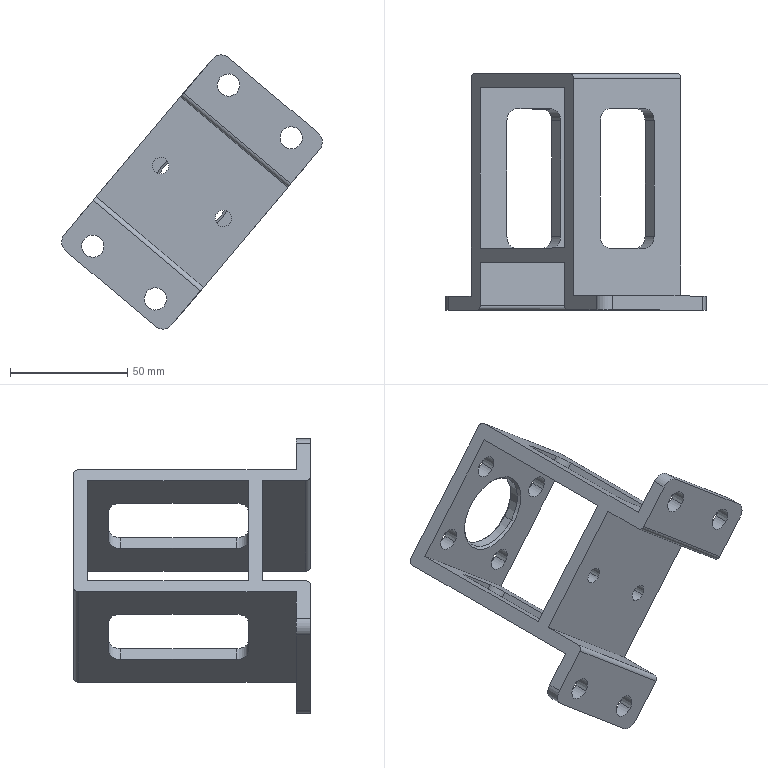Component | SolidWorks | 07FixtureBase-1 | 1 solid | 66 faces | box 111.37 x 101 x 117.17 mm | volume 97150 mm3 | cylinder 38 | plane 24 | cone 4 | commonest cylinder face diameters 9.5 x16 10 x12 7 x4 4 x4 32 x2 | material Aviation Aluminum-7075
build123d program:
from build123d import *

# Parameters (mm, degrees)
BOSS_EXTRUDE1_DEPTH       = 60
CUT_EXTRUDE1_REACH        = 161.578
SKETCH2_R                 = 4.75
CUT_EXTRUDE2_REACH        = 157.849
SKETCH3_R                 = 4.75
FILLET1_R                 = 5
CUT_EXTRUDE3_REACH        = 157.849
SKETCH4_R                 = 16
CUT_EXTRUDE4_DEPTH        = 147.782
BOSS_EXTRUDE2_REACH       = 145.265
SKETCH6_W                 = 60
SKETCH6_H                 = 6
M8X1_0_TAPPED_HOLE1_D     = 7
M8X1_0_TAPPED_HOLE1_DEPTH = 19
M8X1_0_TAPPED_HOLE1_TIP   = 2.103
FILLET2_R                 = 2
CHAMFER1_SIZE             = 1
FILLET3_R                 = 2


with BuildPart() as part:
    # Sketch1 → Boss-Extrude1 (new body)
    with BuildSketch(Plane.XY):
        Polygon((0, 0), (26, 0), (26, -95), (82, -95), (82, 0), (108, 0), (108, -6), (88, -6), (88, -101), (20, -101), (20, -6), (0, -6), align=None)
    extrude(amount=BOSS_EXTRUDE1_DEPTH)

    # Sketch2 → Cut-Extrude1 (cut, up to next)
    with BuildSketch(Plane(origin=(0, 0, 0), x_dir=(1, 0, 0), z_dir=(0, 1, 0)), mode=Mode.PRIVATE) as cut_extrude1_sk1:
        with Locations(Location((9, -12.5, 0), (0, 0, 270))):
            Circle(SKETCH2_R)
    cut_extrude1_tool1 = extrude(cut_extrude1_sk1.sketch, amount=-CUT_EXTRUDE1_REACH, mode=Mode.PRIVATE) & part.part
    # Sketch2 → Cut-Extrude1 (cut, up to next)
    with BuildSketch(Plane(origin=(0, 0, 0), x_dir=(1, 0, 0), z_dir=(0, 1, 0)), mode=Mode.PRIVATE) as cut_extrude1_sk2:
        with Locations(Location((9, -47.5, 0), (0, 0, 270))):
            Circle(SKETCH2_R)
    cut_extrude1_tool2 = extrude(cut_extrude1_sk2.sketch, amount=-CUT_EXTRUDE1_REACH, mode=Mode.PRIVATE) & part.part
    # Sketch2 → Cut-Extrude1 (cut, up to next)
    with BuildSketch(Plane(origin=(0, 0, 0), x_dir=(1, 0, 0), z_dir=(0, 1, 0)), mode=Mode.PRIVATE) as cut_extrude1_sk3:
        with Locations(Location((99, -12.5, 0), (0, 0, 270))):
            Circle(SKETCH2_R)
    cut_extrude1_tool3 = extrude(cut_extrude1_sk3.sketch, amount=-CUT_EXTRUDE1_REACH, mode=Mode.PRIVATE) & part.part
    # Sketch2 → Cut-Extrude1 (cut, up to next)
    with BuildSketch(Plane(origin=(0, 0, 0), x_dir=(1, 0, 0), z_dir=(0, 1, 0)), mode=Mode.PRIVATE) as cut_extrude1_sk4:
        with Locations(Location((99, -47.5, 0), (0, 0, 270))):
            Circle(SKETCH2_R)
    cut_extrude1_tool4 = extrude(cut_extrude1_sk4.sketch, amount=-CUT_EXTRUDE1_REACH, mode=Mode.PRIVATE) & part.part
    add(cut_extrude1_tool1.solids().sort_by_distance((9, 0, 12.5))[0], mode=Mode.SUBTRACT)
    add(cut_extrude1_tool2.solids().sort_by_distance((9, 0, 47.5))[0], mode=Mode.SUBTRACT)
    add(cut_extrude1_tool3.solids().sort_by_distance((99, 0, 12.5))[0], mode=Mode.SUBTRACT)
    add(cut_extrude1_tool4.solids().sort_by_distance((99, 0, 47.5))[0], mode=Mode.SUBTRACT)

    # Sketch3 → Cut-Extrude2 (cut, up to next)
    with BuildSketch(Plane(origin=(0, -95, 0), x_dir=(1, 0, 0), z_dir=(0, 1, 0)), mode=Mode.PRIVATE) as cut_extrude2_sk1:
        with Locations(Location((36.5, -10, 0), (0, 0, 270))):
            Circle(SKETCH3_R)
    cut_extrude2_tool1 = extrude(cut_extrude2_sk1.sketch, amount=-CUT_EXTRUDE2_REACH, mode=Mode.PRIVATE) & part.part
    # Sketch3 → Cut-Extrude2 (cut, up to next)
    with BuildSketch(Plane(origin=(0, -95, 0), x_dir=(1, 0, 0), z_dir=(0, 1, 0)), mode=Mode.PRIVATE) as cut_extrude2_sk2:
        with Locations(Location((71.5, -10, 0), (0, 0, 270))):
            Circle(SKETCH3_R)
    cut_extrude2_tool2 = extrude(cut_extrude2_sk2.sketch, amount=-CUT_EXTRUDE2_REACH, mode=Mode.PRIVATE) & part.part
    # Sketch3 → Cut-Extrude2 (cut, up to next)
    with BuildSketch(Plane(origin=(0, -95, 0), x_dir=(1, 0, 0), z_dir=(0, 1, 0)), mode=Mode.PRIVATE) as cut_extrude2_sk3:
        with Locations(Location((36.5, -50, 0), (0, 0, 270))):
            Circle(SKETCH3_R)
    cut_extrude2_tool3 = extrude(cut_extrude2_sk3.sketch, amount=-CUT_EXTRUDE2_REACH, mode=Mode.PRIVATE) & part.part
    # Sketch3 → Cut-Extrude2 (cut, up to next)
    with BuildSketch(Plane(origin=(0, -95, 0), x_dir=(1, 0, 0), z_dir=(0, 1, 0)), mode=Mode.PRIVATE) as cut_extrude2_sk4:
        with Locations(Location((71.5, -50, 0), (0, 0, 270))):
            Circle(SKETCH3_R)
    cut_extrude2_tool4 = extrude(cut_extrude2_sk4.sketch, amount=-CUT_EXTRUDE2_REACH, mode=Mode.PRIVATE) & part.part
    add(cut_extrude2_tool1.solids().sort_by_distance((36.5, -95, 10))[0], mode=Mode.SUBTRACT)
    add(cut_extrude2_tool2.solids().sort_by_distance((71.5, -95, 10))[0], mode=Mode.SUBTRACT)
    add(cut_extrude2_tool3.solids().sort_by_distance((36.5, -95, 50))[0], mode=Mode.SUBTRACT)
    add(cut_extrude2_tool4.solids().sort_by_distance((71.5, -95, 50))[0], mode=Mode.SUBTRACT)

    # Fillet1
    fillet1_edges = [part.edges().sort_by_distance(p)[0] for p in [
        (108, -3, 0),
        (0, -3, 0),
        (108, -3, 60),
        (0, -3, 60),
    ]]
    fillet(fillet1_edges, radius=FILLET1_R)

    # Sketch4 → Cut-Extrude3 (cut, up to next)
    with BuildSketch(Plane(origin=(0, -95, 0), x_dir=(1, 0, 0), z_dir=(0, 1, 0)), mode=Mode.PRIVATE) as cut_extrude3_sk1:
        with Locations(Location((54, -30, 0), (0, 0, 270))):
            Circle(SKETCH4_R)
    cut_extrude3_tool1 = extrude(cut_extrude3_sk1.sketch, amount=-CUT_EXTRUDE3_REACH, mode=Mode.PRIVATE) & part.part
    add(cut_extrude3_tool1.solids().sort_by_distance((54, -95, 30))[0], mode=Mode.SUBTRACT)

    # Sketch5 → Cut-Extrude4 (cut, through all)
    with BuildSketch(Plane(origin=(88, 0, 0), x_dir=(0, 0, -1), z_dir=(1, 0, 0))):
        with BuildLine():
            Line((-20, -26.5), (-40, -26.5))
            ThreePointArc((-40, -26.5), (-43.536, -27.964), (-45, -31.5))
            Line((-45, -31.5), (-45, -81))
            ThreePointArc((-45, -81), (-43.536, -84.536), (-40, -86))
            Line((-40, -86), (-20, -86))
            ThreePointArc((-20, -86), (-16.464, -84.536), (-15, -81))
            Line((-15, -81), (-15, -31.5))
            ThreePointArc((-15, -31.5), (-16.464, -27.964), (-20, -26.5))
        make_face()
    extrude(amount=-CUT_EXTRUDE4_DEPTH, mode=Mode.SUBTRACT)

    # Sketch6 → Boss-Extrude2 (add, up to next)
    with BuildSketch(Plane(origin=(26, 0, 0), x_dir=(0, 0, -1), z_dir=(1, 0, 0)), mode=Mode.PRIVATE) as boss_extrude2_sk1:
        with Locations((-30, -23.5)):
            Rectangle(SKETCH6_W, SKETCH6_H)
    boss_extrude2_tool1 = extrude(boss_extrude2_sk1.sketch, amount=BOSS_EXTRUDE2_REACH, mode=Mode.PRIVATE) - part.part
    add(boss_extrude2_tool1.solids().sort_by_distance((26, -23.5, 30))[0])

    # M8x1.0 Tapped Hole1
    with Locations(Plane(origin=(54, -20.5, 12.5), x_dir=(1, 0, 0), z_dir=(0, 1, 0))):
        with Locations((0, 0), (0, -35)):
            Hole(M8X1_0_TAPPED_HOLE1_D / 2, depth=M8X1_0_TAPPED_HOLE1_DEPTH)
            with Locations((0, 0, -(M8X1_0_TAPPED_HOLE1_DEPTH + M8X1_0_TAPPED_HOLE1_TIP / 2))):  # 118° drill point
                Cone(0, M8X1_0_TAPPED_HOLE1_D / 2, M8X1_0_TAPPED_HOLE1_TIP, mode=Mode.SUBTRACT)

    # Fillet2
    fillet2_edges = [part.edges().sort_by_distance(p)[0] for p in [
        (88, -101, 30),
        (20, -101, 30),
    ]]
    fillet(fillet2_edges, radius=FILLET2_R)

    # Chamfer1
    chamfer1_edges = [part.edges().sort_by_distance(p)[0] for p in [
        (54, -95, 14),
        (54, -101, 14),
    ]]
    chamfer(chamfer1_edges, length=CHAMFER1_SIZE)

    # Fillet3
    fillet3_edges = [part.edges().sort_by_distance(p)[0] for p in [
        (26, 0, 30),
        (82, 0, 30),
    ]]
    fillet(fillet3_edges, radius=FILLET3_R)


solid = part.part

# Placed as in the assembly
solid = solid.moved(Location((-209.156, 48.645, -139.074), (0, -49.905, -180)))